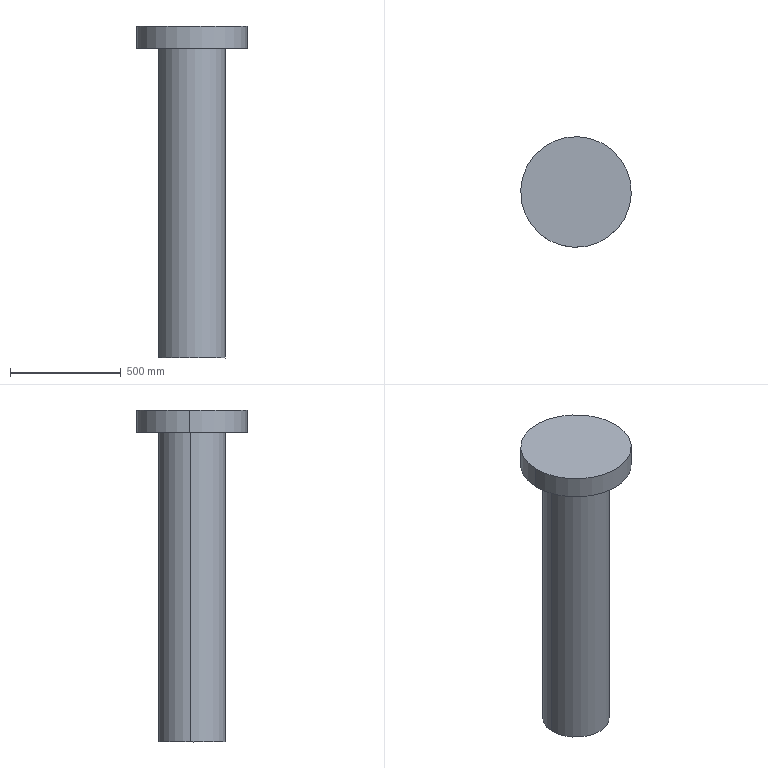Component | SolidWorks | RunningMechanism-5_10-2 | 1 solid | 7 faces | box 500 x 500 x 1500 mm | volume 118595123 mm3 | cylinder 4 | plane 3 | commonest cylinder face diameters 500 x2 300 x2
build123d program:
from build123d import *

# Parameters (mm, degrees)
SKETCH1_R           = 150
BOSS_EXTRUDE1_DEPTH = 725
SKETCH2_R           = 250
BOSS_EXTRUDE2_DEPTH = 50


with BuildPart() as part:
    # Sketch1 → Boss-Extrude1 (new, symmetric)
    with BuildSketch(Plane(origin=(0, 0, 0), x_dir=(0, 0, -1), z_dir=(1, 0, 0))):
        Circle(SKETCH1_R)
    extrude(amount=BOSS_EXTRUDE1_DEPTH, both=True)

    # Sketch2 → Boss-Extrude2 (add, symmetric)
    with BuildSketch(Plane(origin=(725, 0, 0), x_dir=(0, 0, -1), z_dir=(1, 0, 0))):
        Circle(SKETCH2_R)
    extrude(amount=BOSS_EXTRUDE2_DEPTH, both=True)


solid = part.part

# Placed as in the assembly
solid = solid.moved(Location((3141.033, 53898.441, -12001.997), (0, -90, 0)))
STEP:
#1=COLOUR_RGB('',0.7922,0.8196,0.9333);
#2=FILL_AREA_STYLE_COLOUR('',#1);
#3=FILL_AREA_STYLE('',(#2));
#4=SURFACE_STYLE_FILL_AREA(#3);
#5=SURFACE_SIDE_STYLE('',(#4));
#6=SURFACE_STYLE_USAGE(.BOTH.,#5);
#7=PRESENTATION_STYLE_ASSIGNMENT((#6));
#8=CARTESIAN_POINT('',(113.829,2122.398,-442.008));
#9=VERTEX_POINT('',#8);
#10=CARTESIAN_POINT('',(133.497,2121.574,-442.008));
#11=VERTEX_POINT('',#10);
#12=CARTESIAN_POINT('',(123.663,2121.986,-442.008));
#13=DIRECTION('',(0.0000002,0.,1.));
#14=DIRECTION('',(-0.9991,0.04189,0.0000002));
#15=AXIS2_PLACEMENT_3D('',#12,#13,#14);
#16=CIRCLE('',#15,9.843);
#17=EDGE_CURVE('',#9,#11,#16,.T.);
#18=ORIENTED_EDGE('',*,*,#17,.F.);
#19=CARTESIAN_POINT('',(113.829,2122.398,-445.945));
#20=VERTEX_POINT('',#19);
#21=CARTESIAN_POINT('',(113.829,2122.398,-442.008));
#22=DIRECTION('',(-0.0000002,-0.,-1.));
#23=VECTOR('',#22,39.37);
#24=LINE('',#21,#23);
#25=EDGE_CURVE('',#9,#20,#24,.T.);
#26=ORIENTED_EDGE('',*,*,#25,.T.);
#27=CARTESIAN_POINT('',(133.497,2121.574,-445.945));
#28=VERTEX_POINT('',#27);
#29=CARTESIAN_POINT('',(123.663,2121.986,-445.945));
#30=DIRECTION('',(0.0000002,0.,1.));
#31=DIRECTION('',(-0.9991,0.04189,0.0000002));
#32=AXIS2_PLACEMENT_3D('',#29,#30,#31);
#33=CIRCLE('',#32,9.843);
#34=EDGE_CURVE('',#20,#28,#33,.T.);
#35=ORIENTED_EDGE('',*,*,#34,.T.);
#36=CARTESIAN_POINT('',(133.497,2121.574,-442.008));
#37=DIRECTION('',(-0.0000002,-0.,-1.));
#38=VECTOR('',#37,39.37);
#39=LINE('',#36,#38);
#40=EDGE_CURVE('',#11,#28,#39,.T.);
#41=ORIENTED_EDGE('',*,*,#40,.F.);
#42=EDGE_LOOP('',(#18,#26,#35,#41));
#43=FACE_OUTER_BOUND('',#42,.T.);
#44=CARTESIAN_POINT('',(123.663,2121.986,-442.008));
#45=DIRECTION('',(-0.0000002,-0.,-1.));
#46=DIRECTION('',(0.9991,-0.04189,-0.0000002));
#47=AXIS2_PLACEMENT_3D('',#44,#45,#46);
#48=CYLINDRICAL_SURFACE('',#47,9.843);
#49=ADVANCED_FACE('',(#43),#48,.T.);
#50=CARTESIAN_POINT('',(117.762,2122.233,-445.945));
#51=VERTEX_POINT('',#50);
#52=CARTESIAN_POINT('',(129.563,2121.739,-445.945));
#53=VERTEX_POINT('',#52);
#54=CARTESIAN_POINT('',(123.663,2121.986,-445.945));
#55=DIRECTION('',(0.0000002,0.,1.));
#56=DIRECTION('',(-0.9991,0.04189,0.0000002));
#57=AXIS2_PLACEMENT_3D('',#54,#55,#56);
#58=CIRCLE('',#57,5.906);
#59=EDGE_CURVE('',#51,#53,#58,.T.);
#60=ORIENTED_EDGE('',*,*,#59,.F.);
#61=CARTESIAN_POINT('',(117.762,2122.233,-501.063));
#62=VERTEX_POINT('',#61);
#63=CARTESIAN_POINT('',(117.762,2122.233,-443.976));
#64=DIRECTION('',(-0.0000002,-0.,-1.));
#65=VECTOR('',#64,39.37);
#66=LINE('',#63,#65);
#67=EDGE_CURVE('',#51,#62,#66,.T.);
#68=ORIENTED_EDGE('',*,*,#67,.T.);
#69=CARTESIAN_POINT('',(129.563,2121.739,-501.063));
#70=VERTEX_POINT('',#69);
#71=CARTESIAN_POINT('',(123.663,2121.986,-501.063));
#72=DIRECTION('',(0.0000002,0.,1.));
#73=DIRECTION('',(-0.9991,0.04189,0.0000002));
#74=AXIS2_PLACEMENT_3D('',#71,#72,#73);
#75=CIRCLE('',#74,5.906);
#76=EDGE_CURVE('',#62,#70,#75,.T.);
#77=ORIENTED_EDGE('',*,*,#76,.T.);
#78=CARTESIAN_POINT('',(129.563,2121.739,-443.976));
#79=DIRECTION('',(-0.0000002,-0.,-1.));
#80=VECTOR('',#79,39.37);
#81=LINE('',#78,#80);
#82=EDGE_CURVE('',#53,#70,#81,.T.);
#83=ORIENTED_EDGE('',*,*,#82,.F.);
#84=EDGE_LOOP('',(#60,#68,#77,#83));
#85=FACE_OUTER_BOUND('',#84,.T.);
#86=CARTESIAN_POINT('',(123.663,2121.986,-443.976));
#87=DIRECTION('',(-0.0000002,-0.,-1.));
#88=DIRECTION('',(0.9991,-0.04189,-0.0000002));
#89=AXIS2_PLACEMENT_3D('',#86,#87,#88);
#90=CYLINDRICAL_SURFACE('',#89,5.906);
#91=ADVANCED_FACE('',(#85),#90,.T.);
#92=ORIENTED_EDGE('',*,*,#67,.F.);
#93=CARTESIAN_POINT('',(123.663,2121.986,-445.945));
#94=DIRECTION('',(0.0000002,0.,1.));
#95=DIRECTION('',(-0.9991,0.04189,0.0000002));
#96=AXIS2_PLACEMENT_3D('',#93,#94,#95);
#97=CIRCLE('',#96,5.906);
#98=EDGE_CURVE('',#53,#51,#97,.T.);
#99=ORIENTED_EDGE('',*,*,#98,.F.);
#100=ORIENTED_EDGE('',*,*,#82,.T.);
#101=CARTESIAN_POINT('',(123.663,2121.986,-501.063));
#102=DIRECTION('',(0.0000002,0.,1.));
#103=DIRECTION('',(-0.9991,0.04189,0.0000002));
#104=AXIS2_PLACEMENT_3D('',#101,#102,#103);
#105=CIRCLE('',#104,5.906);
#106=EDGE_CURVE('',#70,#62,#105,.T.);
#107=ORIENTED_EDGE('',*,*,#106,.T.);
#108=EDGE_LOOP('',(#92,#99,#100,#107));
#109=FACE_OUTER_BOUND('',#108,.T.);
#110=CARTESIAN_POINT('',(123.663,2121.986,-443.976));
#111=DIRECTION('',(-0.0000002,-0.,-1.));
#112=DIRECTION('',(0.9991,-0.04189,-0.0000002));
#113=AXIS2_PLACEMENT_3D('',#110,#111,#112);
#114=CYLINDRICAL_SURFACE('',#113,5.906);
#115=ADVANCED_FACE('',(#109),#114,.T.);
#116=ORIENTED_EDGE('',*,*,#106,.F.);
#117=ORIENTED_EDGE('',*,*,#76,.F.);
#118=EDGE_LOOP('',(#116,#117));
#119=FACE_OUTER_BOUND('',#118,.T.);
#120=CARTESIAN_POINT('',(123.663,2121.986,-501.063));
#121=DIRECTION('',(0.0000002,0.,1.));
#122=DIRECTION('',(-0.9991,0.04189,0.0000002));
#123=AXIS2_PLACEMENT_3D('',#120,#121,#122);
#124=PLANE('',#123);
#125=ADVANCED_FACE('',(#119),#124,.F.);
#126=ORIENTED_EDGE('',*,*,#25,.F.);
#127=CARTESIAN_POINT('',(123.663,2121.986,-442.008));
#128=DIRECTION('',(0.0000002,0.,1.));
#129=DIRECTION('',(-0.9991,0.04189,0.0000002));
#130=AXIS2_PLACEMENT_3D('',#127,#128,#129);
#131=CIRCLE('',#130,9.843);
#132=EDGE_CURVE('',#11,#9,#131,.T.);
#133=ORIENTED_EDGE('',*,*,#132,.F.);
#134=ORIENTED_EDGE('',*,*,#40,.T.);
#135=CARTESIAN_POINT('',(123.663,2121.986,-445.945));
#136=DIRECTION('',(0.0000002,0.,1.));
#137=DIRECTION('',(-0.9991,0.04189,0.0000002));
#138=AXIS2_PLACEMENT_3D('',#135,#136,#137);
#139=CIRCLE('',#138,9.843);
#140=EDGE_CURVE('',#28,#20,#139,.T.);
#141=ORIENTED_EDGE('',*,*,#140,.T.);
#142=EDGE_LOOP('',(#126,#133,#134,#141));
#143=FACE_OUTER_BOUND('',#142,.T.);
#144=CARTESIAN_POINT('',(123.663,2121.986,-442.008));
#145=DIRECTION('',(-0.0000002,-0.,-1.));
#146=DIRECTION('',(0.9991,-0.04189,-0.0000002));
#147=AXIS2_PLACEMENT_3D('',#144,#145,#146);
#148=CYLINDRICAL_SURFACE('',#147,9.843);
#149=ADVANCED_FACE('',(#143),#148,.T.);
#150=ORIENTED_EDGE('',*,*,#132,.T.);
#151=ORIENTED_EDGE('',*,*,#17,.T.);
#152=EDGE_LOOP('',(#150,#151));
#153=FACE_OUTER_BOUND('',#152,.T.);
#154=CARTESIAN_POINT('',(123.663,2121.986,-442.008));
#155=DIRECTION('',(0.0000002,0.,1.));
#156=DIRECTION('',(-0.9991,0.04189,0.0000002));
#157=AXIS2_PLACEMENT_3D('',#154,#155,#156);
#158=PLANE('',#157);
#159=ADVANCED_FACE('',(#153),#158,.T.);
#160=ORIENTED_EDGE('',*,*,#98,.T.);
#161=ORIENTED_EDGE('',*,*,#59,.T.);
#162=EDGE_LOOP('',(#160,#161));
#163=FACE_BOUND('',#162,.T.);
#164=ORIENTED_EDGE('',*,*,#140,.F.);
#165=ORIENTED_EDGE('',*,*,#34,.F.);
#166=EDGE_LOOP('',(#164,#165));
#167=FACE_OUTER_BOUND('',#166,.T.);
#168=CARTESIAN_POINT('',(123.663,2121.986,-445.945));
#169=DIRECTION('',(0.0000002,0.,1.));
#170=DIRECTION('',(-0.9991,0.04189,0.0000002));
#171=AXIS2_PLACEMENT_3D('',#168,#169,#170);
#172=PLANE('',#171);
#173=ADVANCED_FACE('',(#163,#167),#172,.F.);
#174=CLOSED_SHELL('',(#49,#91,#115,#125,#149,#159,#173));
#175=MANIFOLD_SOLID_BREP('',#174);
#176=STYLED_ITEM('',(#7),#175);
#177=PRESENTATION_LAYER_ASSIGNMENT('','',(#176));
#178=CARTESIAN_POINT('',(0.,0.,0.));
#179=DIRECTION('',(0.,0.,1.));
#180=DIRECTION('',(1.,0.,0.));
#181=AXIS2_PLACEMENT_3D('',#178,#179,#180);
#182=(LENGTH_UNIT()NAMED_UNIT(*)SI_UNIT($,.METRE.));
#183=LENGTH_MEASURE_WITH_UNIT(LENGTH_MEASURE(0.0254),#182);
#184=DIMENSIONAL_EXPONENTS(1.,0.,0.,0.,0.,0.,0.);
#185=(CONVERSION_BASED_UNIT('',#183)LENGTH_UNIT()NAMED_UNIT(#184));
#186=UNCERTAINTY_MEASURE_WITH_UNIT(LENGTH_MEASURE(0.00001),#185,'','');
#187=(NAMED_UNIT(*)PLANE_ANGLE_UNIT()SI_UNIT($,.RADIAN.));
#188=(NAMED_UNIT(*)SI_UNIT($,.STERADIAN.)SOLID_ANGLE_UNIT());
#189=(GEOMETRIC_REPRESENTATION_CONTEXT(3)GLOBAL_UNCERTAINTY_ASSIGNED_CONTEXT((#186))GLOBAL_UNIT_ASSIGNED_CONTEXT((#185,#187,#188))REPRESENTATION_CONTEXT('',''));
#190=ADVANCED_BREP_SHAPE_REPRESENTATION('',(#175,#181),#189);
#191=(LENGTH_UNIT()NAMED_UNIT(*)SI_UNIT($,.METRE.));
#192=LENGTH_MEASURE_WITH_UNIT(LENGTH_MEASURE(0.0254),#191);
#193=DIMENSIONAL_EXPONENTS(1.,0.,0.,0.,0.,0.,0.);
#194=(CONVERSION_BASED_UNIT('',#192)LENGTH_UNIT()NAMED_UNIT(#193));
#195=UNCERTAINTY_MEASURE_WITH_UNIT(LENGTH_MEASURE(0.00001),#194,'','');
#196=(NAMED_UNIT(*)PLANE_ANGLE_UNIT()SI_UNIT($,.RADIAN.));
#197=(NAMED_UNIT(*)SI_UNIT($,.STERADIAN.)SOLID_ANGLE_UNIT());
#198=(GEOMETRIC_REPRESENTATION_CONTEXT(3)GLOBAL_UNCERTAINTY_ASSIGNED_CONTEXT((#195))GLOBAL_UNIT_ASSIGNED_CONTEXT((#194,#196,#197))REPRESENTATION_CONTEXT('',''));
#199=MECHANICAL_DESIGN_GEOMETRIC_PRESENTATION_REPRESENTATION('',(#176),#198);